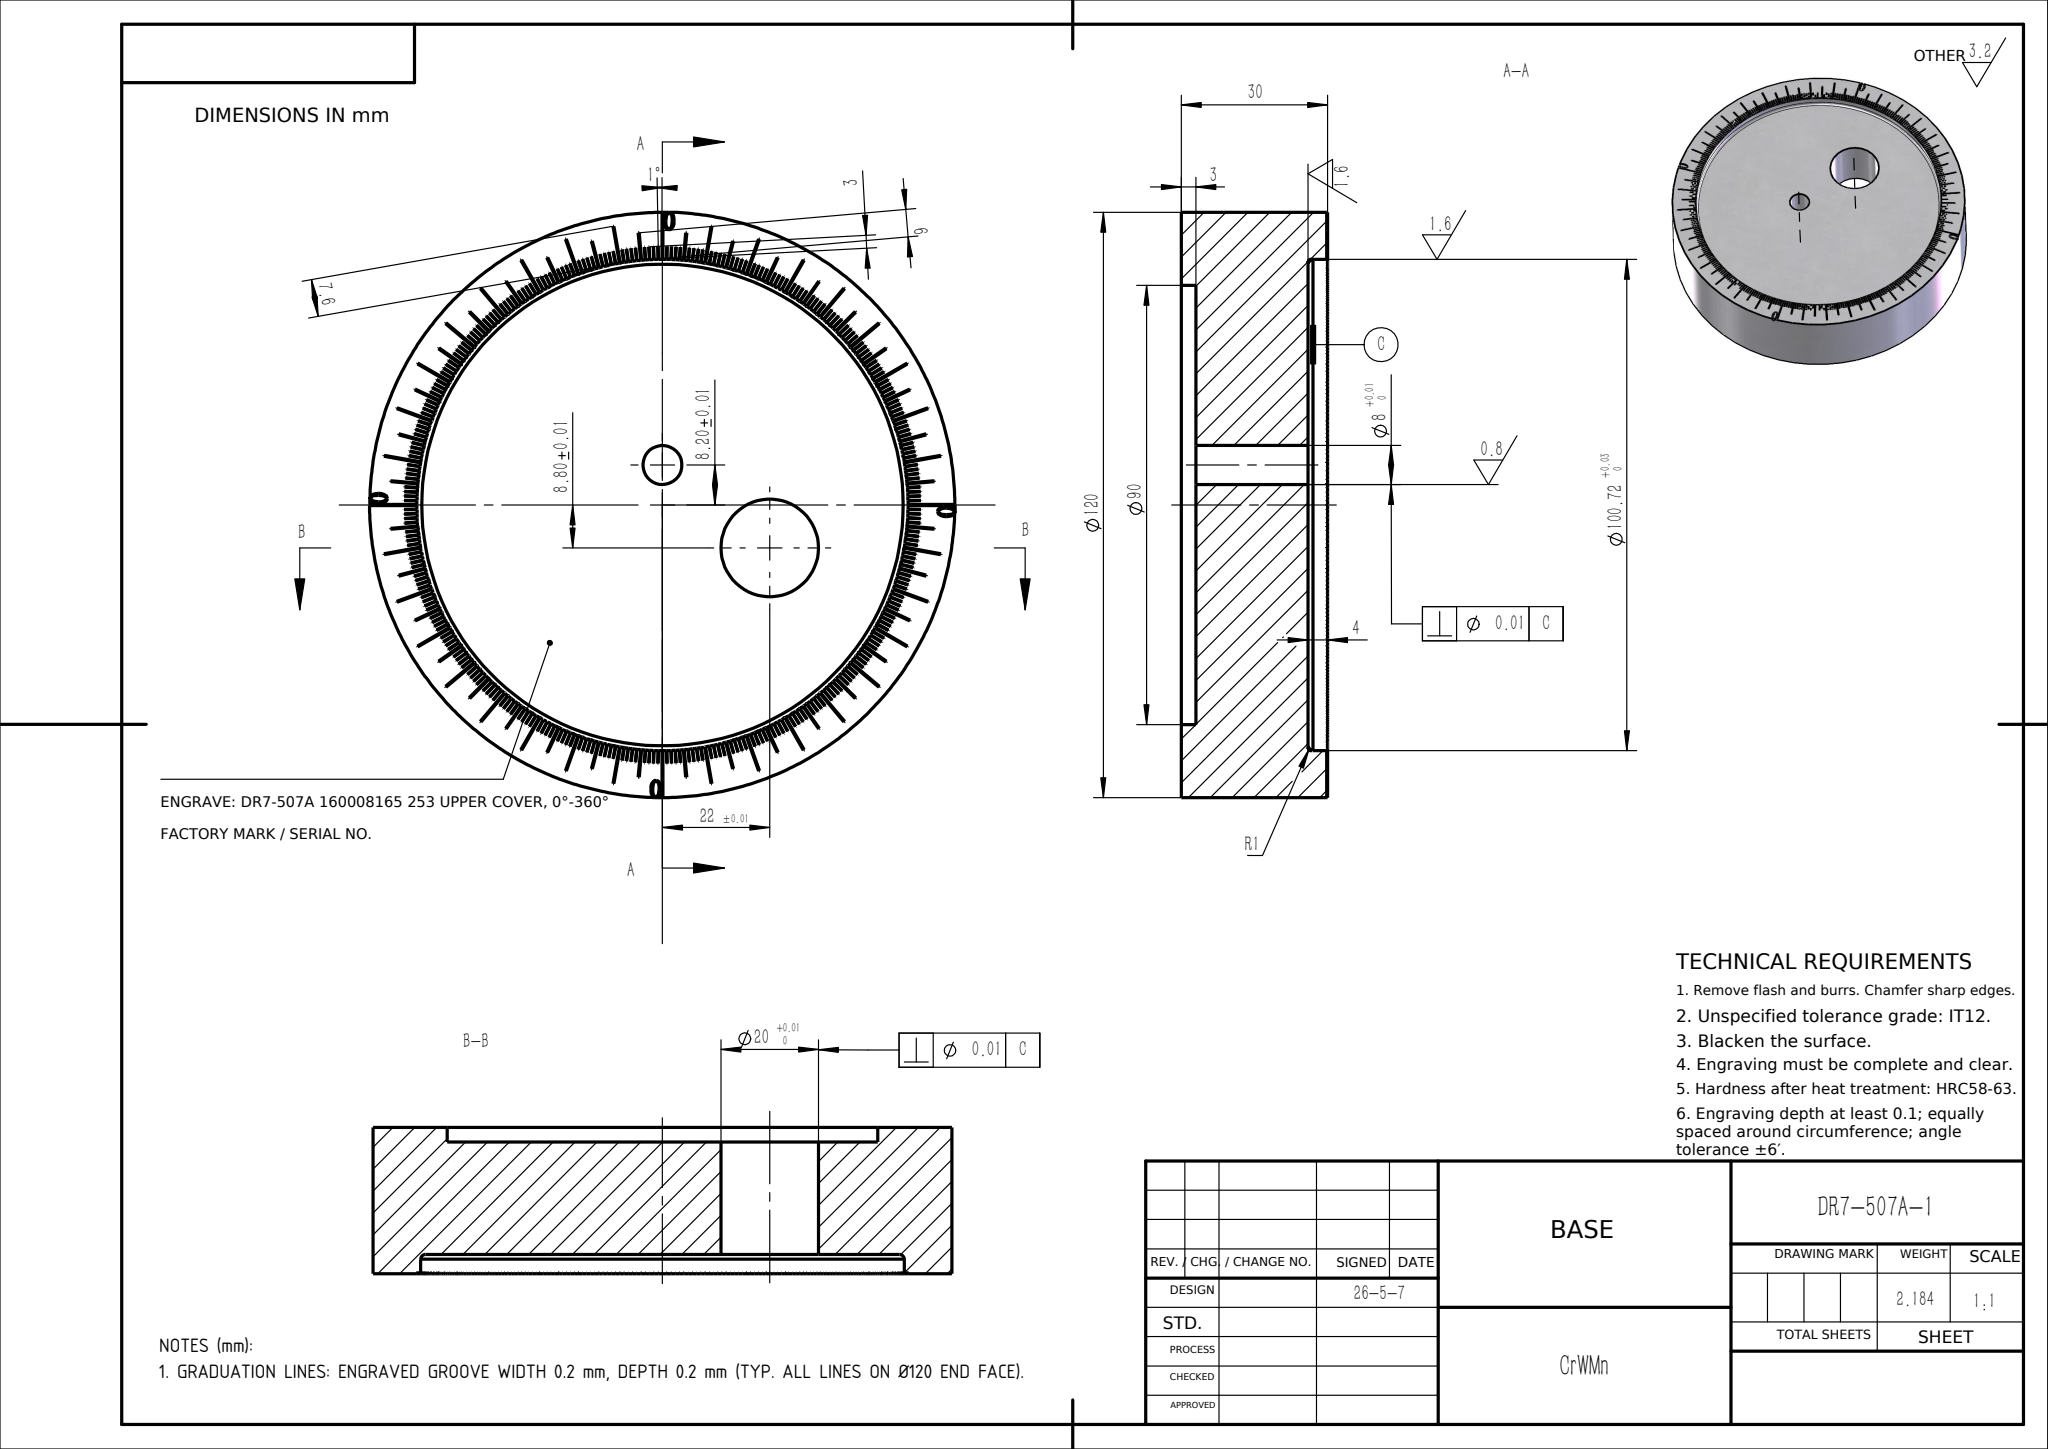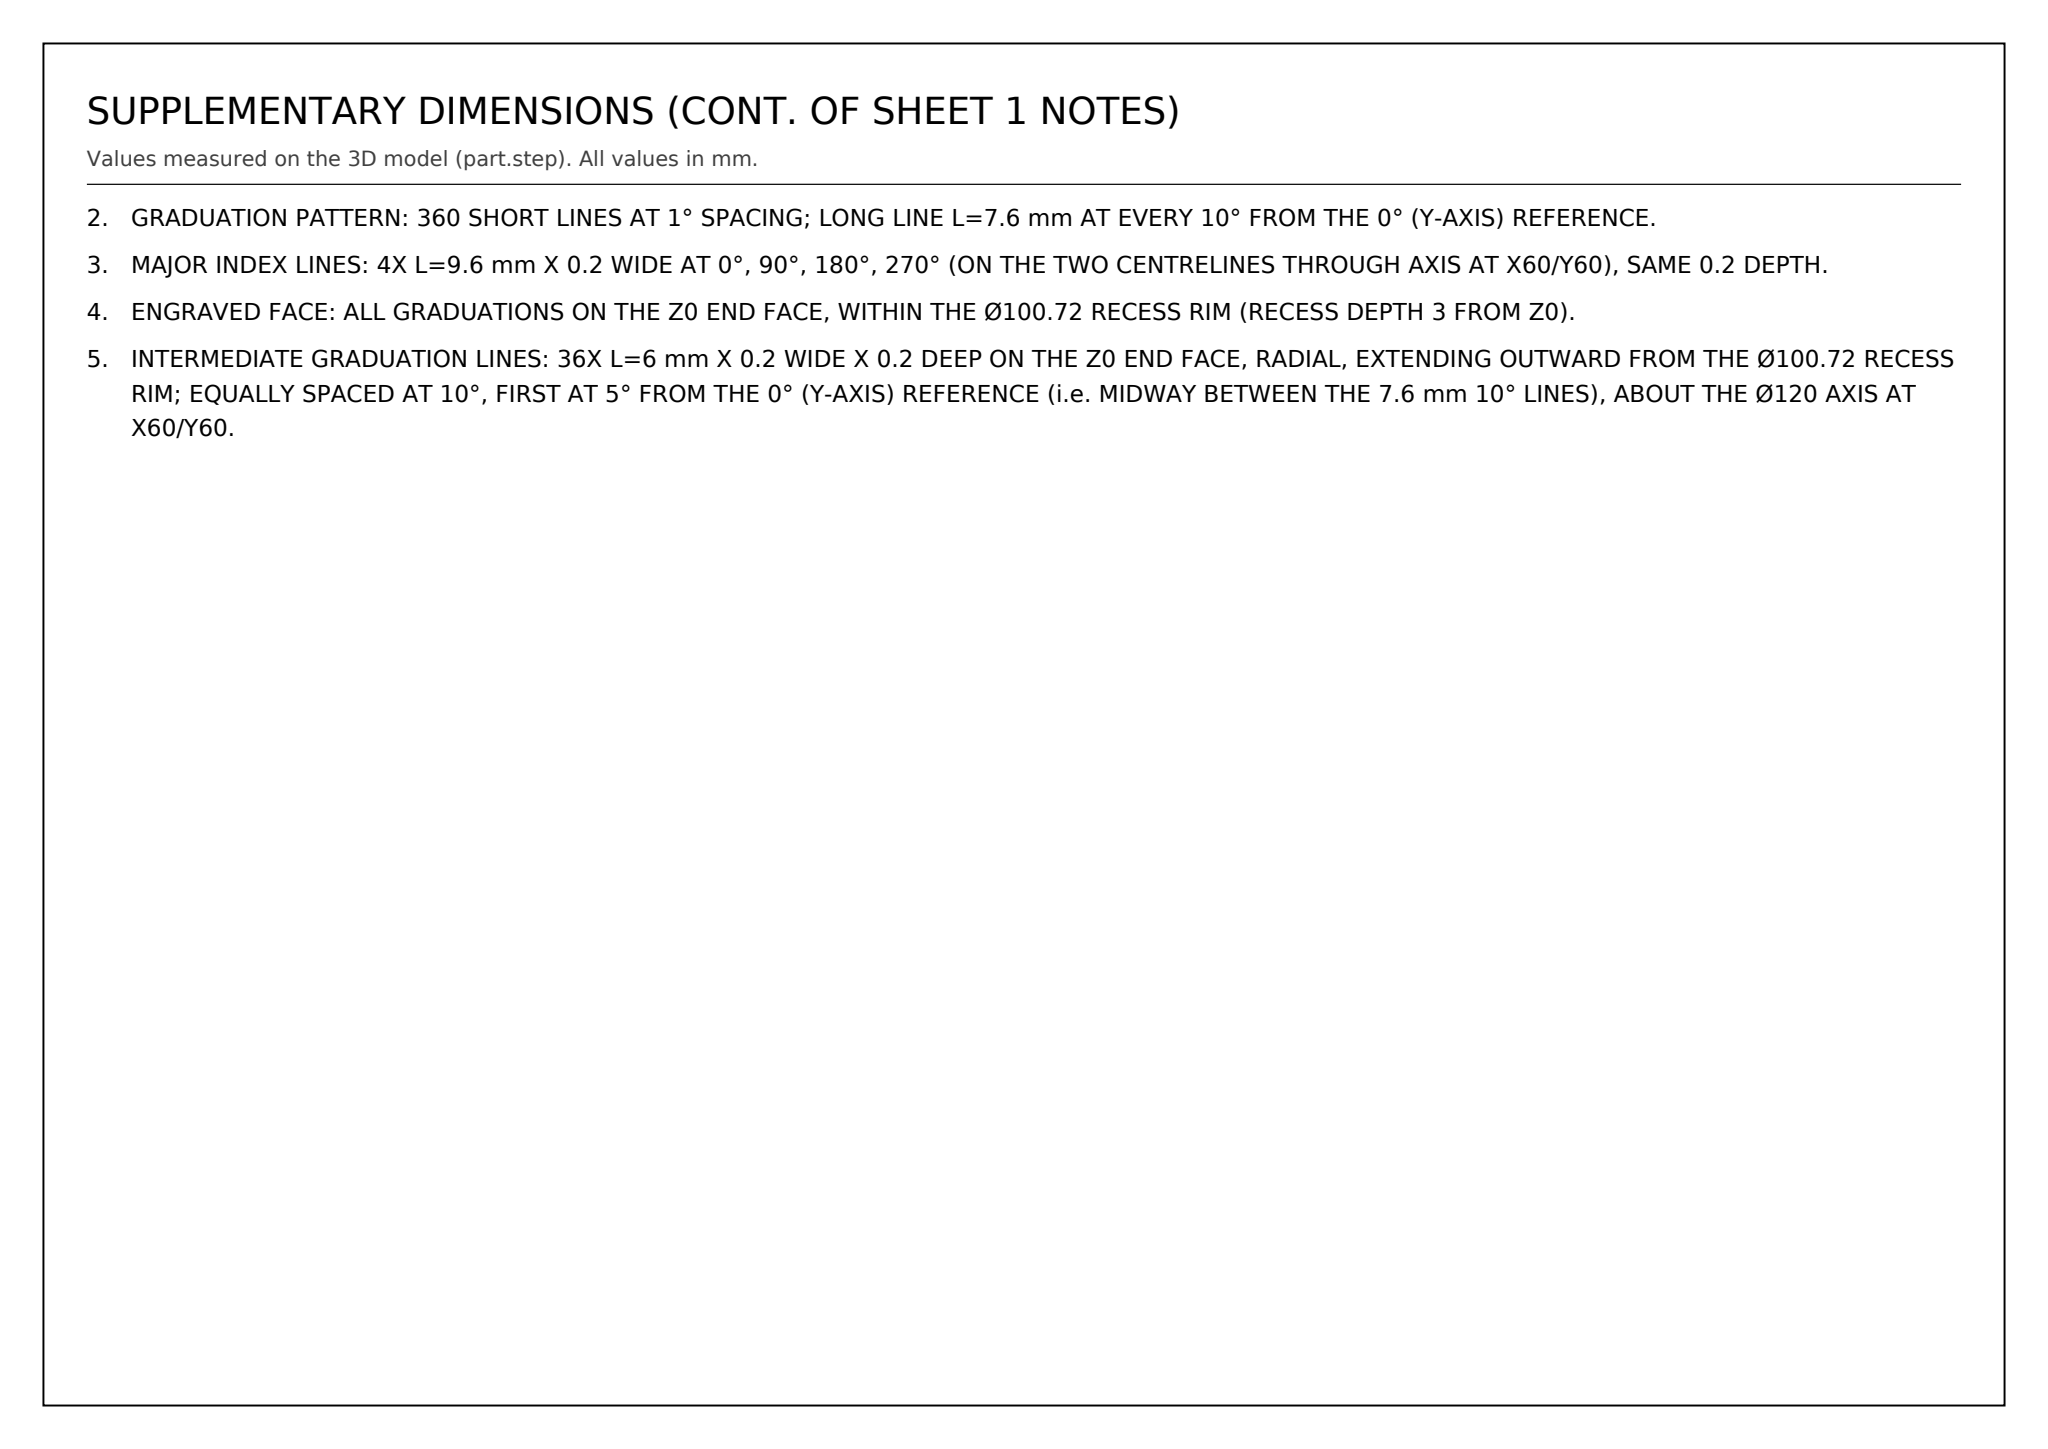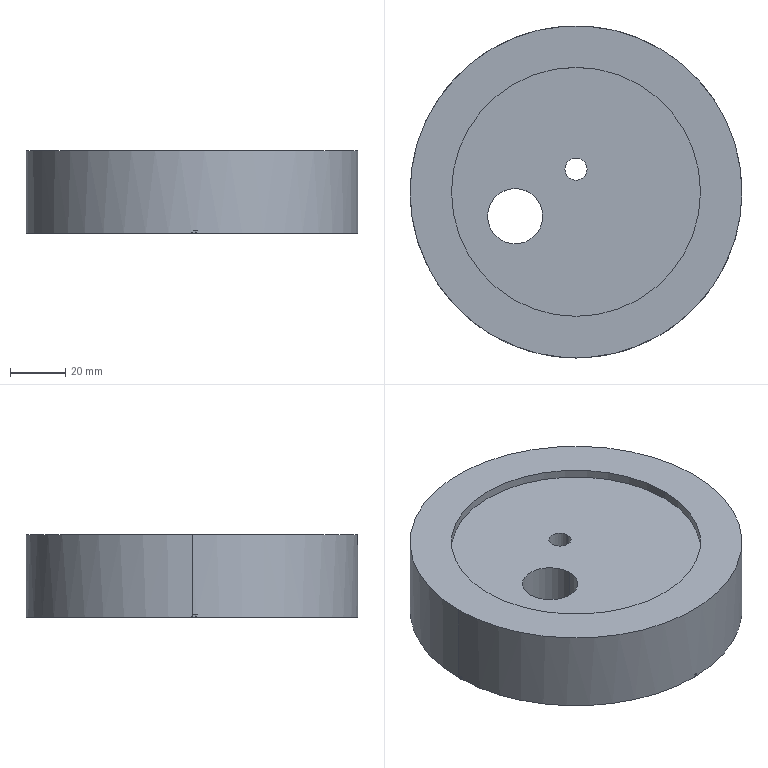Part | SolidWorks | mm | 1 solid | 1495 faces | box 120 x 120 x 30 mm | volume 279978 mm3 | plane 1451 | spline 32 | cylinder 10 | torus 2 | commonest cylinder face diameters 90 x2 120 x2 8 x2 20 x2 100.72 x2
Drawing notes:
GRADUATION LINES: ENGRAVED GROOVE WIDTH 0.2 mm, DEPTH 0.2 mm (TYP. ALL LINES ON Ø120 END FACE). | from the solid: axis_planes normal x at 59.9 and 60.1 (0.2 apart) with z extent [0.0,0.2] forming one graduation groove
GRADUATION PATTERN: 360 SHORT LINES AT 1° SPACING; LONG LINE L=7.6 mm AT EVERY 10° FROM THE 0° (Y-AXIS) REFERENCE. | from the solid: inclined_planes angle_to_xyz_axes [10.0,80.0,90.0], size [1.3,7.5,0.2] (7.6 long mark at 10° increment)
MAJOR INDEX LINES: 4X L=9.6 mm X 0.2 WIDE AT 0°, 90°, 180°, 270° (ON THE TWO CENTRELINES THROUGH AXIS AT X60/Y60), SAME 0.2 DEPTH. | from the solid: axis_planes x=59.9/60.1 with y extents [0.0,9.6] and [110.4,120.0]; y=59.9/60.1 with x extents [0.0,9.6] and [110.4,120.0]
ENGRAVED FACE: ALL GRADUATIONS ON THE Z0 END FACE, WITHIN THE Ø100.72 RECESS RIM (RECESS DEPTH 3 FROM Z0). | from the solid: hole/bore Ø100.72 on z axis at (60,60), from z 0.0 to 3.0; graduation planes at z 0.0-0.2
INTERMEDIATE GRADUATION LINES: 36X L=6 mm X 0.2 WIDE X 0.2 DEEP ON THE Z0 END FACE, RADIAL, EXTENDING OUTWARD FROM THE Ø100.72 RECESS RIM; EQUALLY SPACED AT 10°, FIRST AT 5° FROM THE 0° (Y-AXIS) REFERENCE (i.e. MIDWAY BETWEEN THE 7.6 mm 10° LINES), ABOUT THE Ø120 AXIS AT X60/Y60. | from the solid: axis_planes z=0.2 tick faces, e.g. x[101.2,105.9] y[27.8,31.2] (len 5.8≈6 mm, 125° from +Y) and x[105.6,110.8] y[36.2,38.8] (115°), lying midway between 7.6 mm ticks x[103.6,110.3] y[30.9,34.9] (120°) and x[107.3,114.5] y[77.1,79.9]; inner ends at R50.36 = Ø100.72 bore rim